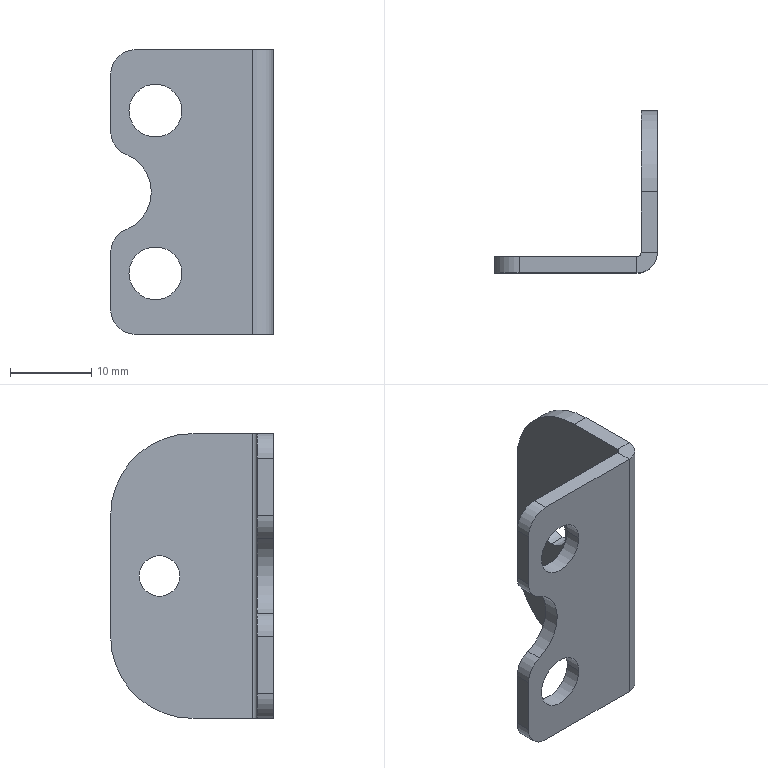Component | SolidWorks | FilmTensionPlate-2 | 1 solid | 28 faces | box 20 x 20 x 35 mm | volume 2267 mm3 | cylinder 15 | plane 13 | commonest cylinder face diameters 6.5 x4 6 x4 5 x3 20 x2 1 x1 10 x1
STEP:
#1=COLOUR_RGB('',0.7922,0.8196,0.9333);
#2=FILL_AREA_STYLE_COLOUR('',#1);
#3=FILL_AREA_STYLE('',(#2));
#4=SURFACE_STYLE_FILL_AREA(#3);
#5=SURFACE_SIDE_STYLE('',(#4));
#6=SURFACE_STYLE_USAGE(.BOTH.,#5);
#7=PRESENTATION_STYLE_ASSIGNMENT((#6));
#8=CARTESIAN_POINT('',(0.9154,-5.709,0.3937));
#9=VERTEX_POINT('',#8);
#10=CARTESIAN_POINT('',(0.6594,-5.709,0.3937));
#11=VERTEX_POINT('',#10);
#12=CARTESIAN_POINT('',(0.7874,-5.709,0.3937));
#13=DIRECTION('',(0.,-1.,0.));
#14=DIRECTION('',(-1.,0.,0.));
#15=AXIS2_PLACEMENT_3D('',#12,#13,#14);
#16=CIRCLE('',#15,0.128);
#17=EDGE_CURVE('',#9,#11,#16,.T.);
#18=ORIENTED_EDGE('',*,*,#17,.F.);
#19=CARTESIAN_POINT('',(0.9154,-5.787,0.3937));
#20=VERTEX_POINT('',#19);
#21=CARTESIAN_POINT('',(0.9154,-5.709,0.3937));
#22=DIRECTION('',(0.,-1.,0.));
#23=VECTOR('',#22,39.37);
#24=LINE('',#21,#23);
#25=EDGE_CURVE('',#9,#20,#24,.T.);
#26=ORIENTED_EDGE('',*,*,#25,.T.);
#27=CARTESIAN_POINT('',(0.6594,-5.787,0.3937));
#28=VERTEX_POINT('',#27);
#29=CARTESIAN_POINT('',(0.7874,-5.787,0.3937));
#30=DIRECTION('',(0.,-1.,0.));
#31=DIRECTION('',(-1.,0.,0.));
#32=AXIS2_PLACEMENT_3D('',#29,#30,#31);
#33=CIRCLE('',#32,0.128);
#34=EDGE_CURVE('',#20,#28,#33,.T.);
#35=ORIENTED_EDGE('',*,*,#34,.T.);
#36=CARTESIAN_POINT('',(0.6594,-5.709,0.3937));
#37=DIRECTION('',(0.,-1.,0.));
#38=VECTOR('',#37,39.37);
#39=LINE('',#36,#38);
#40=EDGE_CURVE('',#11,#28,#39,.T.);
#41=ORIENTED_EDGE('',*,*,#40,.F.);
#42=EDGE_LOOP('',(#18,#26,#35,#41));
#43=FACE_OUTER_BOUND('',#42,.T.);
#44=CARTESIAN_POINT('',(0.7874,-5.709,0.3937));
#45=DIRECTION('',(0.,-1.,0.));
#46=DIRECTION('',(-1.,0.,0.));
#47=AXIS2_PLACEMENT_3D('',#44,#45,#46);
#48=CYLINDRICAL_SURFACE('',#47,0.128);
#49=ADVANCED_FACE('',(#43),#48,.F.);
#50=CARTESIAN_POINT('',(0.9154,-5.709,-0.3937));
#51=VERTEX_POINT('',#50);
#52=CARTESIAN_POINT('',(0.6594,-5.709,-0.3937));
#53=VERTEX_POINT('',#52);
#54=CARTESIAN_POINT('',(0.7874,-5.709,-0.3937));
#55=DIRECTION('',(0.,-1.,0.));
#56=DIRECTION('',(1.,0.,0.));
#57=AXIS2_PLACEMENT_3D('',#54,#55,#56);
#58=CIRCLE('',#57,0.128);
#59=EDGE_CURVE('',#51,#53,#58,.T.);
#60=ORIENTED_EDGE('',*,*,#59,.F.);
#61=CARTESIAN_POINT('',(0.9154,-5.787,-0.3937));
#62=VERTEX_POINT('',#61);
#63=CARTESIAN_POINT('',(0.9154,-5.709,-0.3937));
#64=DIRECTION('',(0.,-1.,0.));
#65=VECTOR('',#64,39.37);
#66=LINE('',#63,#65);
#67=EDGE_CURVE('',#51,#62,#66,.T.);
#68=ORIENTED_EDGE('',*,*,#67,.T.);
#69=CARTESIAN_POINT('',(0.6594,-5.787,-0.3937));
#70=VERTEX_POINT('',#69);
#71=CARTESIAN_POINT('',(0.7874,-5.787,-0.3937));
#72=DIRECTION('',(0.,-1.,0.));
#73=DIRECTION('',(1.,0.,0.));
#74=AXIS2_PLACEMENT_3D('',#71,#72,#73);
#75=CIRCLE('',#74,0.128);
#76=EDGE_CURVE('',#62,#70,#75,.T.);
#77=ORIENTED_EDGE('',*,*,#76,.T.);
#78=CARTESIAN_POINT('',(0.6594,-5.709,-0.3937));
#79=DIRECTION('',(0.,-1.,0.));
#80=VECTOR('',#79,39.37);
#81=LINE('',#78,#80);
#82=EDGE_CURVE('',#53,#70,#81,.T.);
#83=ORIENTED_EDGE('',*,*,#82,.F.);
#84=EDGE_LOOP('',(#60,#68,#77,#83));
#85=FACE_OUTER_BOUND('',#84,.T.);
#86=CARTESIAN_POINT('',(0.7874,-5.709,-0.3937));
#87=DIRECTION('',(0.,-1.,0.));
#88=DIRECTION('',(-1.,0.,0.));
#89=AXIS2_PLACEMENT_3D('',#86,#87,#88);
#90=CYLINDRICAL_SURFACE('',#89,0.128);
#91=ADVANCED_FACE('',(#85),#90,.F.);
#92=CARTESIAN_POINT('',(1.28,-5.236,0.09843));
#93=VERTEX_POINT('',#92);
#94=CARTESIAN_POINT('',(1.28,-5.236,-0.09843));
#95=VERTEX_POINT('',#94);
#96=CARTESIAN_POINT('',(1.28,-5.236,0.));
#97=DIRECTION('',(1.,-0.,0.));
#98=DIRECTION('',(0.,0.,-1.));
#99=AXIS2_PLACEMENT_3D('',#96,#97,#98);
#100=CIRCLE('',#99,0.09843);
#101=EDGE_CURVE('',#93,#95,#100,.T.);
#102=ORIENTED_EDGE('',*,*,#101,.F.);
#103=CARTESIAN_POINT('',(1.358,-5.236,0.09843));
#104=VERTEX_POINT('',#103);
#105=CARTESIAN_POINT('',(1.358,-5.236,0.09843));
#106=DIRECTION('',(1.,-0.,0.));
#107=VECTOR('',#106,39.37);
#108=LINE('',#105,#107);
#109=EDGE_CURVE('',#93,#104,#108,.T.);
#110=ORIENTED_EDGE('',*,*,#109,.T.);
#111=CARTESIAN_POINT('',(1.358,-5.236,-0.09843));
#112=VERTEX_POINT('',#111);
#113=CARTESIAN_POINT('',(1.358,-5.236,0.));
#114=DIRECTION('',(1.,-0.,0.));
#115=DIRECTION('',(0.,0.,-1.));
#116=AXIS2_PLACEMENT_3D('',#113,#114,#115);
#117=CIRCLE('',#116,0.09843);
#118=EDGE_CURVE('',#104,#112,#117,.T.);
#119=ORIENTED_EDGE('',*,*,#118,.T.);
#120=CARTESIAN_POINT('',(1.358,-5.236,-0.09843));
#121=DIRECTION('',(1.,-0.,0.));
#122=VECTOR('',#121,39.37);
#123=LINE('',#120,#122);
#124=EDGE_CURVE('',#95,#112,#123,.T.);
#125=ORIENTED_EDGE('',*,*,#124,.F.);
#126=EDGE_LOOP('',(#102,#110,#119,#125));
#127=FACE_OUTER_BOUND('',#126,.T.);
#128=CARTESIAN_POINT('',(1.358,-5.236,0.));
#129=DIRECTION('',(1.,-0.,0.));
#130=DIRECTION('',(0.,0.,-1.));
#131=AXIS2_PLACEMENT_3D('',#128,#129,#130);
#132=CYLINDRICAL_SURFACE('',#131,0.09843);
#133=ADVANCED_FACE('',(#127),#132,.F.);
#134=CARTESIAN_POINT('',(0.5709,-5.709,0.5709));
#135=VERTEX_POINT('',#134);
#136=CARTESIAN_POINT('',(0.5709,-5.709,0.292));
#137=VERTEX_POINT('',#136);
#138=CARTESIAN_POINT('',(0.5709,-5.709,-0.689));
#139=DIRECTION('',(0.,-0.,-1.));
#140=VECTOR('',#139,39.37);
#141=LINE('',#138,#140);
#142=EDGE_CURVE('',#135,#137,#141,.T.);
#143=ORIENTED_EDGE('',*,*,#142,.T.);
#144=CARTESIAN_POINT('',(0.5709,-5.787,0.292));
#145=VERTEX_POINT('',#144);
#146=CARTESIAN_POINT('',(0.5709,-5.787,0.292));
#147=DIRECTION('',(0.,-1.,0.));
#148=VECTOR('',#147,39.37);
#149=LINE('',#146,#148);
#150=EDGE_CURVE('',#137,#145,#149,.T.);
#151=ORIENTED_EDGE('',*,*,#150,.T.);
#152=CARTESIAN_POINT('',(0.5709,-5.787,0.5709));
#153=VERTEX_POINT('',#152);
#154=CARTESIAN_POINT('',(0.5709,-5.787,0.));
#155=DIRECTION('',(0.,-0.,-1.));
#156=VECTOR('',#155,39.37);
#157=LINE('',#154,#156);
#158=EDGE_CURVE('',#153,#145,#157,.T.);
#159=ORIENTED_EDGE('',*,*,#158,.F.);
#160=CARTESIAN_POINT('',(0.5709,-5.787,0.5709));
#161=DIRECTION('',(-0.,1.,-0.));
#162=VECTOR('',#161,39.37);
#163=LINE('',#160,#162);
#164=EDGE_CURVE('',#153,#135,#163,.T.);
#165=ORIENTED_EDGE('',*,*,#164,.T.);
#166=EDGE_LOOP('',(#143,#151,#159,#165));
#167=FACE_OUTER_BOUND('',#166,.T.);
#168=CARTESIAN_POINT('',(0.5709,-5.787,-0.689));
#169=DIRECTION('',(1.,0.,-0.));
#170=DIRECTION('',(0.,-1.,0.));
#171=AXIS2_PLACEMENT_3D('',#168,#169,#170);
#172=PLANE('',#171);
#173=ADVANCED_FACE('',(#167),#172,.F.);
#174=CARTESIAN_POINT('',(1.358,-5.394,0.689));
#175=VERTEX_POINT('',#174);
#176=CARTESIAN_POINT('',(1.358,-5.689,0.689));
#177=VERTEX_POINT('',#176);
#178=CARTESIAN_POINT('',(1.358,-5.,0.689));
#179=DIRECTION('',(-0.,-1.,0.));
#180=VECTOR('',#179,39.37);
#181=LINE('',#178,#180);
#182=EDGE_CURVE('',#175,#177,#181,.T.);
#183=ORIENTED_EDGE('',*,*,#182,.F.);
#184=CARTESIAN_POINT('',(1.28,-5.394,0.689));
#185=VERTEX_POINT('',#184);
#186=CARTESIAN_POINT('',(1.28,-5.394,0.689));
#187=DIRECTION('',(-1.,0.,-0.));
#188=VECTOR('',#187,39.37);
#189=LINE('',#186,#188);
#190=EDGE_CURVE('',#175,#185,#189,.T.);
#191=ORIENTED_EDGE('',*,*,#190,.T.);
#192=CARTESIAN_POINT('',(1.28,-5.689,0.689));
#193=VERTEX_POINT('',#192);
#194=CARTESIAN_POINT('',(1.28,-5.,0.689));
#195=DIRECTION('',(-0.,-1.,0.));
#196=VECTOR('',#195,39.37);
#197=LINE('',#194,#196);
#198=EDGE_CURVE('',#185,#193,#197,.T.);
#199=ORIENTED_EDGE('',*,*,#198,.T.);
#200=CARTESIAN_POINT('',(1.28,-5.689,0.689));
#201=DIRECTION('',(1.,-0.,0.));
#202=VECTOR('',#201,39.37);
#203=LINE('',#200,#202);
#204=EDGE_CURVE('',#193,#177,#203,.T.);
#205=ORIENTED_EDGE('',*,*,#204,.T.);
#206=EDGE_LOOP('',(#183,#191,#199,#205));
#207=FACE_OUTER_BOUND('',#206,.T.);
#208=CARTESIAN_POINT('',(1.28,-5.,0.689));
#209=DIRECTION('',(-0.,0.,1.));
#210=DIRECTION('',(-0.,-1.,0.));
#211=AXIS2_PLACEMENT_3D('',#208,#209,#210);
#212=PLANE('',#211);
#213=ADVANCED_FACE('',(#207),#212,.T.);
#214=CARTESIAN_POINT('',(1.28,-5.236,0.));
#215=DIRECTION('',(1.,-0.,0.));
#216=DIRECTION('',(0.,0.,-1.));
#217=AXIS2_PLACEMENT_3D('',#214,#215,#216);
#218=CIRCLE('',#217,0.09843);
#219=EDGE_CURVE('',#95,#93,#218,.T.);
#220=ORIENTED_EDGE('',*,*,#219,.T.);
#221=ORIENTED_EDGE('',*,*,#101,.T.);
#222=EDGE_LOOP('',(#220,#221));
#223=FACE_BOUND('',#222,.T.);
#224=CARTESIAN_POINT('',(1.28,-5.,-0.2953));
#225=VERTEX_POINT('',#224);
#226=CARTESIAN_POINT('',(1.28,-5.,0.2953));
#227=VERTEX_POINT('',#226);
#228=CARTESIAN_POINT('',(1.28,-5.,0.689));
#229=DIRECTION('',(0.,0.,1.));
#230=VECTOR('',#229,39.37);
#231=LINE('',#228,#230);
#232=EDGE_CURVE('',#225,#227,#231,.T.);
#233=ORIENTED_EDGE('',*,*,#232,.F.);
#234=CARTESIAN_POINT('',(1.28,-5.394,-0.689));
#235=VERTEX_POINT('',#234);
#236=CARTESIAN_POINT('',(1.28,-5.394,-0.2953));
#237=DIRECTION('',(-1.,0.,-0.));
#238=DIRECTION('',(0.,0.,-1.));
#239=AXIS2_PLACEMENT_3D('',#236,#237,#238);
#240=CIRCLE('',#239,0.3937);
#241=EDGE_CURVE('',#225,#235,#240,.T.);
#242=ORIENTED_EDGE('',*,*,#241,.T.);
#243=CARTESIAN_POINT('',(1.28,-5.689,-0.689));
#244=VERTEX_POINT('',#243);
#245=CARTESIAN_POINT('',(1.28,-5.,-0.689));
#246=DIRECTION('',(0.,1.,-0.));
#247=VECTOR('',#246,39.37);
#248=LINE('',#245,#247);
#249=EDGE_CURVE('',#244,#235,#248,.T.);
#250=ORIENTED_EDGE('',*,*,#249,.F.);
#251=CARTESIAN_POINT('',(1.28,-5.689,0.689));
#252=DIRECTION('',(0.,-0.,-1.));
#253=VECTOR('',#252,39.37);
#254=LINE('',#251,#253);
#255=EDGE_CURVE('',#193,#244,#254,.T.);
#256=ORIENTED_EDGE('',*,*,#255,.F.);
#257=ORIENTED_EDGE('',*,*,#198,.F.);
#258=CARTESIAN_POINT('',(1.28,-5.394,0.2953));
#259=DIRECTION('',(-1.,0.,-0.));
#260=DIRECTION('',(0.,0.,-1.));
#261=AXIS2_PLACEMENT_3D('',#258,#259,#260);
#262=CIRCLE('',#261,0.3937);
#263=EDGE_CURVE('',#185,#227,#262,.T.);
#264=ORIENTED_EDGE('',*,*,#263,.T.);
#265=EDGE_LOOP('',(#233,#242,#250,#256,#257,#264));
#266=FACE_OUTER_BOUND('',#265,.T.);
#267=CARTESIAN_POINT('',(1.28,-5.394,0.));
#268=DIRECTION('',(1.,-0.,0.));
#269=DIRECTION('',(0.,-0.,-1.));
#270=AXIS2_PLACEMENT_3D('',#267,#268,#269);
#271=PLANE('',#270);
#272=ADVANCED_FACE('',(#223,#266),#271,.F.);
#273=CARTESIAN_POINT('',(1.358,-5.236,0.));
#274=DIRECTION('',(1.,-0.,0.));
#275=DIRECTION('',(0.,0.,-1.));
#276=AXIS2_PLACEMENT_3D('',#273,#274,#275);
#277=CIRCLE('',#276,0.09843);
#278=EDGE_CURVE('',#112,#104,#277,.T.);
#279=ORIENTED_EDGE('',*,*,#278,.F.);
#280=ORIENTED_EDGE('',*,*,#118,.F.);
#281=EDGE_LOOP('',(#279,#280));
#282=FACE_BOUND('',#281,.T.);
#283=CARTESIAN_POINT('',(1.358,-5.689,-0.689));
#284=VERTEX_POINT('',#283);
#285=CARTESIAN_POINT('',(1.358,-5.394,-0.689));
#286=VERTEX_POINT('',#285);
#287=CARTESIAN_POINT('',(1.358,-5.,-0.689));
#288=DIRECTION('',(0.,1.,-0.));
#289=VECTOR('',#288,39.37);
#290=LINE('',#287,#289);
#291=EDGE_CURVE('',#284,#286,#290,.T.);
#292=ORIENTED_EDGE('',*,*,#291,.T.);
#293=CARTESIAN_POINT('',(1.358,-5.,-0.2953));
#294=VERTEX_POINT('',#293);
#295=CARTESIAN_POINT('',(1.358,-5.394,-0.2953));
#296=DIRECTION('',(1.,-0.,0.));
#297=DIRECTION('',(0.,0.,-1.));
#298=AXIS2_PLACEMENT_3D('',#295,#296,#297);
#299=CIRCLE('',#298,0.3937);
#300=EDGE_CURVE('',#286,#294,#299,.T.);
#301=ORIENTED_EDGE('',*,*,#300,.T.);
#302=CARTESIAN_POINT('',(1.358,-5.,0.2953));
#303=VERTEX_POINT('',#302);
#304=CARTESIAN_POINT('',(1.358,-5.,0.689));
#305=DIRECTION('',(0.,0.,1.));
#306=VECTOR('',#305,39.37);
#307=LINE('',#304,#306);
#308=EDGE_CURVE('',#294,#303,#307,.T.);
#309=ORIENTED_EDGE('',*,*,#308,.T.);
#310=CARTESIAN_POINT('',(1.358,-5.394,0.2953));
#311=DIRECTION('',(1.,-0.,0.));
#312=DIRECTION('',(0.,0.,-1.));
#313=AXIS2_PLACEMENT_3D('',#310,#311,#312);
#314=CIRCLE('',#313,0.3937);
#315=EDGE_CURVE('',#303,#175,#314,.T.);
#316=ORIENTED_EDGE('',*,*,#315,.T.);
#317=ORIENTED_EDGE('',*,*,#182,.T.);
#318=CARTESIAN_POINT('',(1.358,-5.689,0.689));
#319=DIRECTION('',(0.,-0.,-1.));
#320=VECTOR('',#319,39.37);
#321=LINE('',#318,#320);
#322=EDGE_CURVE('',#177,#284,#321,.T.);
#323=ORIENTED_EDGE('',*,*,#322,.T.);
#324=EDGE_LOOP('',(#292,#301,#309,#316,#317,#323));
#325=FACE_OUTER_BOUND('',#324,.T.);
#326=CARTESIAN_POINT('',(1.358,-5.394,0.));
#327=DIRECTION('',(1.,-0.,0.));
#328=DIRECTION('',(0.,-0.,-1.));
#329=AXIS2_PLACEMENT_3D('',#326,#327,#328);
#330=PLANE('',#329);
#331=ADVANCED_FACE('',(#282,#325),#330,.T.);
#332=ORIENTED_EDGE('',*,*,#249,.T.);
#333=CARTESIAN_POINT('',(1.28,-5.394,-0.689));
#334=DIRECTION('',(1.,-0.,0.));
#335=VECTOR('',#334,39.37);
#336=LINE('',#333,#335);
#337=EDGE_CURVE('',#235,#286,#336,.T.);
#338=ORIENTED_EDGE('',*,*,#337,.T.);
#339=ORIENTED_EDGE('',*,*,#291,.F.);
#340=CARTESIAN_POINT('',(1.28,-5.689,-0.689));
#341=DIRECTION('',(1.,-0.,0.));
#342=VECTOR('',#341,39.37);
#343=LINE('',#340,#342);
#344=EDGE_CURVE('',#244,#284,#343,.T.);
#345=ORIENTED_EDGE('',*,*,#344,.F.);
#346=EDGE_LOOP('',(#332,#338,#339,#345));
#347=FACE_OUTER_BOUND('',#346,.T.);
#348=CARTESIAN_POINT('',(1.28,-5.,-0.689));
#349=DIRECTION('',(0.,-0.,-1.));
#350=DIRECTION('',(0.,1.,-0.));
#351=AXIS2_PLACEMENT_3D('',#348,#349,#350);
#352=PLANE('',#351);
#353=ADVANCED_FACE('',(#347),#352,.T.);
#354=ORIENTED_EDGE('',*,*,#308,.F.);
#355=CARTESIAN_POINT('',(1.28,-5.,-0.2953));
#356=DIRECTION('',(-1.,0.,-0.));
#357=VECTOR('',#356,39.37);
#358=LINE('',#355,#357);
#359=EDGE_CURVE('',#294,#225,#358,.T.);
#360=ORIENTED_EDGE('',*,*,#359,.T.);
#361=ORIENTED_EDGE('',*,*,#232,.T.);
#362=CARTESIAN_POINT('',(1.28,-5.,0.2953));
#363=DIRECTION('',(1.,-0.,0.));
#364=VECTOR('',#363,39.37);
#365=LINE('',#362,#364);
#366=EDGE_CURVE('',#227,#303,#365,.T.);
#367=ORIENTED_EDGE('',*,*,#366,.T.);
#368=EDGE_LOOP('',(#354,#360,#361,#367));
#369=FACE_OUTER_BOUND('',#368,.T.);
#370=CARTESIAN_POINT('',(1.28,-5.,0.689));
#371=DIRECTION('',(0.,1.,-0.));
#372=DIRECTION('',(1.,-0.,0.));
#373=AXIS2_PLACEMENT_3D('',#370,#371,#372);
#374=PLANE('',#373);
#375=ADVANCED_FACE('',(#369),#374,.T.);
#376=CARTESIAN_POINT('',(1.26,-5.709,-0.689));
#377=VERTEX_POINT('',#376);
#378=CARTESIAN_POINT('',(1.26,-5.787,-0.689));
#379=VERTEX_POINT('',#378);
#380=CARTESIAN_POINT('',(1.26,-5.787,-0.689));
#381=DIRECTION('',(0.,-1.,0.));
#382=VECTOR('',#381,39.37);
#383=LINE('',#380,#382);
#384=EDGE_CURVE('',#377,#379,#383,.T.);
#385=ORIENTED_EDGE('',*,*,#384,.F.);
#386=CARTESIAN_POINT('',(1.26,-5.689,-0.689));
#387=DIRECTION('',(0.,-0.,-1.));
#388=DIRECTION('',(1.,0.,0.));
#389=AXIS2_PLACEMENT_3D('',#386,#387,#388);
#390=CIRCLE('',#389,0.01969);
#391=EDGE_CURVE('',#244,#377,#390,.T.);
#392=ORIENTED_EDGE('',*,*,#391,.F.);
#393=ORIENTED_EDGE('',*,*,#344,.T.);
#394=CARTESIAN_POINT('',(1.26,-5.689,-0.689));
#395=DIRECTION('',(0.,-0.,-1.));
#396=DIRECTION('',(1.,-0.,0.));
#397=AXIS2_PLACEMENT_3D('',#394,#395,#396);
#398=CIRCLE('',#397,0.09843);
#399=EDGE_CURVE('',#284,#379,#398,.T.);
#400=ORIENTED_EDGE('',*,*,#399,.T.);
#401=EDGE_LOOP('',(#385,#392,#393,#400));
#402=FACE_OUTER_BOUND('',#401,.T.);
#403=CARTESIAN_POINT('',(1.26,-5.689,-0.689));
#404=DIRECTION('',(0.,-0.,-1.));
#405=DIRECTION('',(-1.,0.,-0.));
#406=AXIS2_PLACEMENT_3D('',#403,#404,#405);
#407=PLANE('',#406);
#408=ADVANCED_FACE('',(#402),#407,.T.);
#409=CARTESIAN_POINT('',(1.26,-5.709,0.689));
#410=VERTEX_POINT('',#409);
#411=CARTESIAN_POINT('',(1.26,-5.689,0.689));
#412=DIRECTION('',(0.,0.,1.));
#413=DIRECTION('',(1.,0.,0.));
#414=AXIS2_PLACEMENT_3D('',#411,#412,#413);
#415=CIRCLE('',#414,0.01969);
#416=EDGE_CURVE('',#410,#193,#415,.T.);
#417=ORIENTED_EDGE('',*,*,#416,.F.);
#418=CARTESIAN_POINT('',(1.26,-5.787,0.689));
#419=VERTEX_POINT('',#418);
#420=CARTESIAN_POINT('',(1.26,-5.709,0.689));
#421=DIRECTION('',(0.,-1.,0.));
#422=VECTOR('',#421,39.37);
#423=LINE('',#420,#422);
#424=EDGE_CURVE('',#410,#419,#423,.T.);
#425=ORIENTED_EDGE('',*,*,#424,.T.);
#426=CARTESIAN_POINT('',(1.26,-5.689,0.689));
#427=DIRECTION('',(0.,0.,1.));
#428=DIRECTION('',(1.,0.,0.));
#429=AXIS2_PLACEMENT_3D('',#426,#427,#428);
#430=CIRCLE('',#429,0.09843);
#431=EDGE_CURVE('',#419,#177,#430,.T.);
#432=ORIENTED_EDGE('',*,*,#431,.T.);
#433=ORIENTED_EDGE('',*,*,#204,.F.);
#434=EDGE_LOOP('',(#417,#425,#432,#433));
#435=FACE_OUTER_BOUND('',#434,.T.);
#436=CARTESIAN_POINT('',(1.26,-5.689,0.689));
#437=DIRECTION('',(0.,-0.,-1.));
#438=DIRECTION('',(-1.,0.,-0.));
#439=AXIS2_PLACEMENT_3D('',#436,#437,#438);
#440=PLANE('',#439);
#441=ADVANCED_FACE('',(#435),#440,.F.);
#442=ORIENTED_EDGE('',*,*,#322,.F.);
#443=ORIENTED_EDGE('',*,*,#431,.F.);
#444=CARTESIAN_POINT('',(1.26,-5.787,-0.689));
#445=DIRECTION('',(0.,-0.,-1.));
#446=VECTOR('',#445,39.37);
#447=LINE('',#444,#446);
#448=EDGE_CURVE('',#419,#379,#447,.T.);
#449=ORIENTED_EDGE('',*,*,#448,.T.);
#450=ORIENTED_EDGE('',*,*,#399,.F.);
#451=EDGE_LOOP('',(#442,#443,#449,#450));
#452=FACE_OUTER_BOUND('',#451,.T.);
#453=CARTESIAN_POINT('',(1.26,-5.689,0.689));
#454=DIRECTION('',(0.,0.,1.));
#455=DIRECTION('',(0.,-1.,0.));
#456=AXIS2_PLACEMENT_3D('',#453,#454,#455);
#457=CYLINDRICAL_SURFACE('',#456,0.09843);
#458=ADVANCED_FACE('',(#452),#457,.T.);
#459=ORIENTED_EDGE('',*,*,#255,.T.);
#460=ORIENTED_EDGE('',*,*,#391,.T.);
#461=CARTESIAN_POINT('',(1.26,-5.709,-0.689));
#462=DIRECTION('',(0.,0.,1.));
#463=VECTOR('',#462,39.37);
#464=LINE('',#461,#463);
#465=EDGE_CURVE('',#377,#410,#464,.T.);
#466=ORIENTED_EDGE('',*,*,#465,.T.);
#467=ORIENTED_EDGE('',*,*,#416,.T.);
#468=EDGE_LOOP('',(#459,#460,#466,#467));
#469=FACE_OUTER_BOUND('',#468,.T.);
#470=CARTESIAN_POINT('',(1.26,-5.689,0.689));
#471=DIRECTION('',(0.,0.,1.));
#472=DIRECTION('',(0.,-1.,0.));
#473=AXIS2_PLACEMENT_3D('',#470,#471,#472);
#474=CYLINDRICAL_SURFACE('',#473,0.01969);
#475=ADVANCED_FACE('',(#469),#474,.F.);
#476=CARTESIAN_POINT('',(0.689,-5.709,0.689));
#477=VERTEX_POINT('',#476);
#478=CARTESIAN_POINT('',(0.5709,-5.709,0.689));
#479=DIRECTION('',(-1.,-0.,-0.));
#480=VECTOR('',#479,39.37);
#481=LINE('',#478,#480);
#482=EDGE_CURVE('',#410,#477,#481,.T.);
#483=ORIENTED_EDGE('',*,*,#482,.T.);
#484=CARTESIAN_POINT('',(0.689,-5.787,0.689));
#485=VERTEX_POINT('',#484);
#486=CARTESIAN_POINT('',(0.689,-5.787,0.689));
#487=DIRECTION('',(0.,-1.,0.));
#488=VECTOR('',#487,39.37);
#489=LINE('',#486,#488);
#490=EDGE_CURVE('',#477,#485,#489,.T.);
#491=ORIENTED_EDGE('',*,*,#490,.T.);
#492=CARTESIAN_POINT('',(1.358,-5.787,0.689));
#493=DIRECTION('',(-1.,-0.,-0.));
#494=VECTOR('',#493,39.37);
#495=LINE('',#492,#494);
#496=EDGE_CURVE('',#419,#485,#495,.T.);
#497=ORIENTED_EDGE('',*,*,#496,.F.);
#498=ORIENTED_EDGE('',*,*,#424,.F.);
#499=EDGE_LOOP('',(#483,#491,#497,#498));
#500=FACE_OUTER_BOUND('',#499,.T.);
#501=CARTESIAN_POINT('',(0.5709,-5.787,0.689));
#502=DIRECTION('',(0.,-0.,-1.));
#503=DIRECTION('',(-1.,0.,-0.));
#504=AXIS2_PLACEMENT_3D('',#501,#502,#503);
#505=PLANE('',#504);
#506=ADVANCED_FACE('',(#500),#505,.F.);
#507=CARTESIAN_POINT('',(0.689,-5.787,-0.689));
#508=VERTEX_POINT('',#507);
#509=CARTESIAN_POINT('',(1.358,-5.787,-0.689));
#510=DIRECTION('',(1.,0.,-0.));
#511=VECTOR('',#510,39.37);
#512=LINE('',#509,#511);
#513=EDGE_CURVE('',#508,#379,#512,.T.);
#514=ORIENTED_EDGE('',*,*,#513,.F.);
#515=CARTESIAN_POINT('',(0.689,-5.709,-0.689));
#516=VERTEX_POINT('',#515);
#517=CARTESIAN_POINT('',(0.689,-5.787,-0.689));
#518=DIRECTION('',(-0.,1.,-0.));
#519=VECTOR('',#518,39.37);
#520=LINE('',#517,#519);
#521=EDGE_CURVE('',#508,#516,#520,.T.);
#522=ORIENTED_EDGE('',*,*,#521,.T.);
#523=CARTESIAN_POINT('',(1.28,-5.709,-0.689));
#524=DIRECTION('',(1.,0.,-0.));
#525=VECTOR('',#524,39.37);
#526=LINE('',#523,#525);
#527=EDGE_CURVE('',#516,#377,#526,.T.);
#528=ORIENTED_EDGE('',*,*,#527,.T.);
#529=ORIENTED_EDGE('',*,*,#384,.T.);
#530=EDGE_LOOP('',(#514,#522,#528,#529));
#531=FACE_OUTER_BOUND('',#530,.T.);
#532=CARTESIAN_POINT('',(1.28,-5.787,-0.689));
#533=DIRECTION('',(-0.,0.,1.));
#534=DIRECTION('',(1.,-0.,0.));
#535=AXIS2_PLACEMENT_3D('',#532,#533,#534);
#536=PLANE('',#535);
#537=ADVANCED_FACE('',(#531),#536,.F.);
#538=CARTESIAN_POINT('',(0.7874,-5.787,0.3937));
#539=DIRECTION('',(0.,-1.,0.));
#540=DIRECTION('',(-1.,0.,0.));
#541=AXIS2_PLACEMENT_3D('',#538,#539,#540);
#542=CIRCLE('',#541,0.128);
#543=EDGE_CURVE('',#28,#20,#542,.T.);
#544=ORIENTED_EDGE('',*,*,#543,.F.);
#545=ORIENTED_EDGE('',*,*,#34,.F.);
#546=EDGE_LOOP('',(#544,#545));
#547=FACE_BOUND('',#546,.T.);
#548=CARTESIAN_POINT('',(0.7874,-5.787,-0.3937));
#549=DIRECTION('',(0.,-1.,0.));
#550=DIRECTION('',(1.,0.,0.));
#551=AXIS2_PLACEMENT_3D('',#548,#549,#550);
#552=CIRCLE('',#551,0.128);
#553=EDGE_CURVE('',#70,#62,#552,.T.);
#554=ORIENTED_EDGE('',*,*,#553,.F.);
#555=ORIENTED_EDGE('',*,*,#76,.F.);
#556=EDGE_LOOP('',(#554,#555));
#557=FACE_BOUND('',#556,.T.);
#558=CARTESIAN_POINT('',(0.5709,-5.787,-0.292));
#559=VERTEX_POINT('',#558);
#560=CARTESIAN_POINT('',(0.5709,-5.787,-0.5709));
#561=VERTEX_POINT('',#560);
#562=CARTESIAN_POINT('',(0.5709,-5.787,0.));
#563=DIRECTION('',(0.,-0.,-1.));
#564=VECTOR('',#563,39.37);
#565=LINE('',#562,#564);
#566=EDGE_CURVE('',#559,#561,#565,.T.);
#567=ORIENTED_EDGE('',*,*,#566,.T.);
#568=CARTESIAN_POINT('',(0.689,-5.787,-0.5709));
#569=DIRECTION('',(0.,-1.,0.));
#570=DIRECTION('',(1.,0.,0.));
#571=AXIS2_PLACEMENT_3D('',#568,#569,#570);
#572=CIRCLE('',#571,0.1181);
#573=EDGE_CURVE('',#561,#508,#572,.T.);
#574=ORIENTED_EDGE('',*,*,#573,.T.);
#575=ORIENTED_EDGE('',*,*,#513,.T.);
#576=ORIENTED_EDGE('',*,*,#448,.F.);
#577=ORIENTED_EDGE('',*,*,#496,.T.);
#578=CARTESIAN_POINT('',(0.689,-5.787,0.5709));
#579=DIRECTION('',(0.,-1.,0.));
#580=DIRECTION('',(1.,0.,0.));
#581=AXIS2_PLACEMENT_3D('',#578,#579,#580);
#582=CIRCLE('',#581,0.1181);
#583=EDGE_CURVE('',#485,#153,#582,.T.);
#584=ORIENTED_EDGE('',*,*,#583,.T.);
#585=ORIENTED_EDGE('',*,*,#158,.T.);
#586=CARTESIAN_POINT('',(0.6447,-5.787,0.1825));
#587=VERTEX_POINT('',#586);
#588=CARTESIAN_POINT('',(0.689,-5.787,0.292));
#589=DIRECTION('',(0.,-1.,0.));
#590=DIRECTION('',(1.,0.,0.));
#591=AXIS2_PLACEMENT_3D('',#588,#589,#590);
#592=CIRCLE('',#591,0.1181);
#593=EDGE_CURVE('',#145,#587,#592,.T.);
#594=ORIENTED_EDGE('',*,*,#593,.T.);
#595=CARTESIAN_POINT('',(0.6447,-5.787,-0.1825));
#596=VERTEX_POINT('',#595);
#597=CARTESIAN_POINT('',(0.5709,-5.787,0.));
#598=DIRECTION('',(0.,-1.,0.));
#599=DIRECTION('',(-1.,0.,0.));
#600=AXIS2_PLACEMENT_3D('',#597,#598,#599);
#601=CIRCLE('',#600,0.1969);
#602=EDGE_CURVE('',#596,#587,#601,.T.);
#603=ORIENTED_EDGE('',*,*,#602,.F.);
#604=CARTESIAN_POINT('',(0.689,-5.787,-0.292));
#605=DIRECTION('',(0.,-1.,0.));
#606=DIRECTION('',(1.,0.,-0.));
#607=AXIS2_PLACEMENT_3D('',#604,#605,#606);
#608=CIRCLE('',#607,0.1181);
#609=EDGE_CURVE('',#596,#559,#608,.T.);
#610=ORIENTED_EDGE('',*,*,#609,.T.);
#611=EDGE_LOOP('',(#567,#574,#575,#576,#577,#584,#585,#594,#603,#610));
#612=FACE_OUTER_BOUND('',#611,.T.);
#613=CARTESIAN_POINT('',(1.358,-5.787,0.));
#614=DIRECTION('',(-0.,1.,-0.));
#615=DIRECTION('',(1.,0.,-0.));
#616=AXIS2_PLACEMENT_3D('',#613,#614,#615);
#617=PLANE('',#616);
#618=ADVANCED_FACE('',(#547,#557,#612),#617,.F.);
#619=CARTESIAN_POINT('',(0.7874,-5.709,0.3937));
#620=DIRECTION('',(0.,-1.,0.));
#621=DIRECTION('',(-1.,0.,0.));
#622=AXIS2_PLACEMENT_3D('',#619,#620,#621);
#623=CIRCLE('',#622,0.128);
#624=EDGE_CURVE('',#11,#9,#623,.T.);
#625=ORIENTED_EDGE('',*,*,#624,.T.);
#626=ORIENTED_EDGE('',*,*,#17,.T.);
#627=EDGE_LOOP('',(#625,#626));
#628=FACE_BOUND('',#627,.T.);
#629=CARTESIAN_POINT('',(0.7874,-5.709,-0.3937));
#630=DIRECTION('',(0.,-1.,0.));
#631=DIRECTION('',(1.,0.,0.));
#632=AXIS2_PLACEMENT_3D('',#629,#630,#631);
#633=CIRCLE('',#632,0.128);
#634=EDGE_CURVE('',#53,#51,#633,.T.);
#635=ORIENTED_EDGE('',*,*,#634,.T.);
#636=ORIENTED_EDGE('',*,*,#59,.T.);
#637=EDGE_LOOP('',(#635,#636));
#638=FACE_BOUND('',#637,.T.);
#639=ORIENTED_EDGE('',*,*,#527,.F.);
#640=CARTESIAN_POINT('',(0.5709,-5.709,-0.5709));
#641=VERTEX_POINT('',#640);
#642=CARTESIAN_POINT('',(0.689,-5.709,-0.5709));
#643=DIRECTION('',(-0.,1.,-0.));
#644=DIRECTION('',(1.,0.,0.));
#645=AXIS2_PLACEMENT_3D('',#642,#643,#644);
#646=CIRCLE('',#645,0.1181);
#647=EDGE_CURVE('',#516,#641,#646,.T.);
#648=ORIENTED_EDGE('',*,*,#647,.T.);
#649=CARTESIAN_POINT('',(0.5709,-5.709,-0.292));
#650=VERTEX_POINT('',#649);
#651=CARTESIAN_POINT('',(0.5709,-5.709,-0.689));
#652=DIRECTION('',(0.,-0.,-1.));
#653=VECTOR('',#652,39.37);
#654=LINE('',#651,#653);
#655=EDGE_CURVE('',#650,#641,#654,.T.);
#656=ORIENTED_EDGE('',*,*,#655,.F.);
#657=CARTESIAN_POINT('',(0.6447,-5.709,-0.1825));
#658=VERTEX_POINT('',#657);
#659=CARTESIAN_POINT('',(0.689,-5.709,-0.292));
#660=DIRECTION('',(-0.,1.,-0.));
#661=DIRECTION('',(1.,0.,0.));
#662=AXIS2_PLACEMENT_3D('',#659,#660,#661);
#663=CIRCLE('',#662,0.1181);
#664=EDGE_CURVE('',#650,#658,#663,.T.);
#665=ORIENTED_EDGE('',*,*,#664,.T.);
#666=CARTESIAN_POINT('',(0.6447,-5.709,0.1825));
#667=VERTEX_POINT('',#666);
#668=CARTESIAN_POINT('',(0.5709,-5.709,0.));
#669=DIRECTION('',(0.,-1.,0.));
#670=DIRECTION('',(-1.,0.,0.));
#671=AXIS2_PLACEMENT_3D('',#668,#669,#670);
#672=CIRCLE('',#671,0.1969);
#673=EDGE_CURVE('',#658,#667,#672,.T.);
#674=ORIENTED_EDGE('',*,*,#673,.T.);
#675=CARTESIAN_POINT('',(0.689,-5.709,0.292));
#676=DIRECTION('',(-0.,1.,-0.));
#677=DIRECTION('',(1.,0.,0.));
#678=AXIS2_PLACEMENT_3D('',#675,#676,#677);
#679=CIRCLE('',#678,0.1181);
#680=EDGE_CURVE('',#667,#137,#679,.T.);
#681=ORIENTED_EDGE('',*,*,#680,.T.);
#682=ORIENTED_EDGE('',*,*,#142,.F.);
#683=CARTESIAN_POINT('',(0.689,-5.709,0.5709));
#684=DIRECTION('',(-0.,1.,-0.));
#685=DIRECTION('',(1.,0.,0.));
#686=AXIS2_PLACEMENT_3D('',#683,#684,#685);
#687=CIRCLE('',#686,0.1181);
#688=EDGE_CURVE('',#135,#477,#687,.T.);
#689=ORIENTED_EDGE('',*,*,#688,.T.);
#690=ORIENTED_EDGE('',*,*,#482,.F.);
#691=ORIENTED_EDGE('',*,*,#465,.F.);
#692=EDGE_LOOP('',(#639,#648,#656,#665,#674,#681,#682,#689,#690,#691));
#693=FACE_OUTER_BOUND('',#692,.T.);
#694=CARTESIAN_POINT('',(1.358,-5.709,0.));
#695=DIRECTION('',(-0.,1.,-0.));
#696=DIRECTION('',(1.,0.,-0.));
#697=AXIS2_PLACEMENT_3D('',#694,#695,#696);
#698=PLANE('',#697);
#699=ADVANCED_FACE('',(#628,#638,#693),#698,.T.);
#700=ORIENTED_EDGE('',*,*,#655,.T.);
#701=CARTESIAN_POINT('',(0.5709,-5.787,-0.5709));
#702=DIRECTION('',(0.,-1.,0.));
#703=VECTOR('',#702,39.37);
#704=LINE('',#701,#703);
#705=EDGE_CURVE('',#641,#561,#704,.T.);
#706=ORIENTED_EDGE('',*,*,#705,.T.);
#707=ORIENTED_EDGE('',*,*,#566,.F.);
#708=CARTESIAN_POINT('',(0.5709,-5.787,-0.292));
#709=DIRECTION('',(-0.,1.,-0.));
#710=VECTOR('',#709,39.37);
#711=LINE('',#708,#710);
#712=EDGE_CURVE('',#559,#650,#711,.T.);
#713=ORIENTED_EDGE('',*,*,#712,.T.);
#714=EDGE_LOOP('',(#700,#706,#707,#713));
#715=FACE_OUTER_BOUND('',#714,.T.);
#716=CARTESIAN_POINT('',(0.5709,-5.787,-0.689));
#717=DIRECTION('',(1.,0.,-0.));
#718=DIRECTION('',(0.,-1.,0.));
#719=AXIS2_PLACEMENT_3D('',#716,#717,#718);
#720=PLANE('',#719);
#721=ADVANCED_FACE('',(#715),#720,.F.);
#722=ORIENTED_EDGE('',*,*,#109,.F.);
#723=ORIENTED_EDGE('',*,*,#219,.F.);
#724=ORIENTED_EDGE('',*,*,#124,.T.);
#725=ORIENTED_EDGE('',*,*,#278,.T.);
#726=EDGE_LOOP('',(#722,#723,#724,#725));
#727=FACE_OUTER_BOUND('',#726,.T.);
#728=CARTESIAN_POINT('',(1.358,-5.236,0.));
#729=DIRECTION('',(1.,-0.,0.));
#730=DIRECTION('',(0.,0.,-1.));
#731=AXIS2_PLACEMENT_3D('',#728,#729,#730);
#732=CYLINDRICAL_SURFACE('',#731,0.09843);
#733=ADVANCED_FACE('',(#727),#732,.F.);
#734=ORIENTED_EDGE('',*,*,#241,.F.);
#735=ORIENTED_EDGE('',*,*,#359,.F.);
#736=ORIENTED_EDGE('',*,*,#300,.F.);
#737=ORIENTED_EDGE('',*,*,#337,.F.);
#738=EDGE_LOOP('',(#734,#735,#736,#737));
#739=FACE_OUTER_BOUND('',#738,.T.);
#740=CARTESIAN_POINT('',(1.28,-5.394,-0.2953));
#741=DIRECTION('',(1.,-0.,0.));
#742=DIRECTION('',(0.,0.,-1.));
#743=AXIS2_PLACEMENT_3D('',#740,#741,#742);
#744=CYLINDRICAL_SURFACE('',#743,0.3937);
#745=ADVANCED_FACE('',(#739),#744,.T.);
#746=ORIENTED_EDGE('',*,*,#263,.F.);
#747=ORIENTED_EDGE('',*,*,#190,.F.);
#748=ORIENTED_EDGE('',*,*,#315,.F.);
#749=ORIENTED_EDGE('',*,*,#366,.F.);
#750=EDGE_LOOP('',(#746,#747,#748,#749));
#751=FACE_OUTER_BOUND('',#750,.T.);
#752=CARTESIAN_POINT('',(1.28,-5.394,0.2953));
#753=DIRECTION('',(1.,-0.,0.));
#754=DIRECTION('',(0.,0.,-1.));
#755=AXIS2_PLACEMENT_3D('',#752,#753,#754);
#756=CYLINDRICAL_SURFACE('',#755,0.3937);
#757=ADVANCED_FACE('',(#751),#756,.T.);
#758=ORIENTED_EDGE('',*,*,#673,.F.);
#759=CARTESIAN_POINT('',(0.6447,-5.709,-0.1825));
#760=DIRECTION('',(0.,-1.,0.));
#761=VECTOR('',#760,39.37);
#762=LINE('',#759,#761);
#763=EDGE_CURVE('',#658,#596,#762,.T.);
#764=ORIENTED_EDGE('',*,*,#763,.T.);
#765=ORIENTED_EDGE('',*,*,#602,.T.);
#766=CARTESIAN_POINT('',(0.6447,-5.709,0.1825));
#767=DIRECTION('',(-0.,1.,-0.));
#768=VECTOR('',#767,39.37);
#769=LINE('',#766,#768);
#770=EDGE_CURVE('',#587,#667,#769,.T.);
#771=ORIENTED_EDGE('',*,*,#770,.T.);
#772=EDGE_LOOP('',(#758,#764,#765,#771));
#773=FACE_OUTER_BOUND('',#772,.T.);
#774=CARTESIAN_POINT('',(0.5709,-5.709,0.));
#775=DIRECTION('',(0.,-1.,0.));
#776=DIRECTION('',(-1.,0.,0.));
#777=AXIS2_PLACEMENT_3D('',#774,#775,#776);
#778=CYLINDRICAL_SURFACE('',#777,0.1969);
#779=ADVANCED_FACE('',(#773),#778,.F.);
#780=ORIENTED_EDGE('',*,*,#67,.F.);
#781=ORIENTED_EDGE('',*,*,#634,.F.);
#782=ORIENTED_EDGE('',*,*,#82,.T.);
#783=ORIENTED_EDGE('',*,*,#553,.T.);
#784=EDGE_LOOP('',(#780,#781,#782,#783));
#785=FACE_OUTER_BOUND('',#784,.T.);
#786=CARTESIAN_POINT('',(0.7874,-5.709,-0.3937));
#787=DIRECTION('',(0.,-1.,0.));
#788=DIRECTION('',(-1.,0.,0.));
#789=AXIS2_PLACEMENT_3D('',#786,#787,#788);
#790=CYLINDRICAL_SURFACE('',#789,0.128);
#791=ADVANCED_FACE('',(#785),#790,.F.);
#792=ORIENTED_EDGE('',*,*,#25,.F.);
#793=ORIENTED_EDGE('',*,*,#624,.F.);
#794=ORIENTED_EDGE('',*,*,#40,.T.);
#795=ORIENTED_EDGE('',*,*,#543,.T.);
#796=EDGE_LOOP('',(#792,#793,#794,#795));
#797=FACE_OUTER_BOUND('',#796,.T.);
#798=CARTESIAN_POINT('',(0.7874,-5.709,0.3937));
#799=DIRECTION('',(0.,-1.,0.));
#800=DIRECTION('',(-1.,0.,0.));
#801=AXIS2_PLACEMENT_3D('',#798,#799,#800);
#802=CYLINDRICAL_SURFACE('',#801,0.128);
#803=ADVANCED_FACE('',(#797),#802,.F.);
#804=ORIENTED_EDGE('',*,*,#573,.F.);
#805=ORIENTED_EDGE('',*,*,#705,.F.);
#806=ORIENTED_EDGE('',*,*,#647,.F.);
#807=ORIENTED_EDGE('',*,*,#521,.F.);
#808=EDGE_LOOP('',(#804,#805,#806,#807));
#809=FACE_OUTER_BOUND('',#808,.T.);
#810=CARTESIAN_POINT('',(0.689,-5.787,-0.5709));
#811=DIRECTION('',(-0.,1.,-0.));
#812=DIRECTION('',(1.,0.,0.));
#813=AXIS2_PLACEMENT_3D('',#810,#811,#812);
#814=CYLINDRICAL_SURFACE('',#813,0.1181);
#815=ADVANCED_FACE('',(#809),#814,.T.);
#816=ORIENTED_EDGE('',*,*,#609,.F.);
#817=ORIENTED_EDGE('',*,*,#763,.F.);
#818=ORIENTED_EDGE('',*,*,#664,.F.);
#819=ORIENTED_EDGE('',*,*,#712,.F.);
#820=EDGE_LOOP('',(#816,#817,#818,#819));
#821=FACE_OUTER_BOUND('',#820,.T.);
#822=CARTESIAN_POINT('',(0.689,-5.709,-0.292));
#823=DIRECTION('',(0.,-1.,0.));
#824=DIRECTION('',(-1.,0.,0.));
#825=AXIS2_PLACEMENT_3D('',#822,#823,#824);
#826=CYLINDRICAL_SURFACE('',#825,0.1181);
#827=ADVANCED_FACE('',(#821),#826,.T.);
#828=ORIENTED_EDGE('',*,*,#680,.F.);
#829=ORIENTED_EDGE('',*,*,#770,.F.);
#830=ORIENTED_EDGE('',*,*,#593,.F.);
#831=ORIENTED_EDGE('',*,*,#150,.F.);
#832=EDGE_LOOP('',(#828,#829,#830,#831));
#833=FACE_OUTER_BOUND('',#832,.T.);
#834=CARTESIAN_POINT('',(0.689,-5.709,0.292));
#835=DIRECTION('',(0.,-1.,0.));
#836=DIRECTION('',(-1.,0.,0.));
#837=AXIS2_PLACEMENT_3D('',#834,#835,#836);
#838=CYLINDRICAL_SURFACE('',#837,0.1181);
#839=ADVANCED_FACE('',(#833),#838,.T.);
#840=ORIENTED_EDGE('',*,*,#583,.F.);
#841=ORIENTED_EDGE('',*,*,#490,.F.);
#842=ORIENTED_EDGE('',*,*,#688,.F.);
#843=ORIENTED_EDGE('',*,*,#164,.F.);
#844=EDGE_LOOP('',(#840,#841,#842,#843));
#845=FACE_OUTER_BOUND('',#844,.T.);
#846=CARTESIAN_POINT('',(0.689,-5.787,0.5709));
#847=DIRECTION('',(-0.,1.,-0.));
#848=DIRECTION('',(1.,0.,0.));
#849=AXIS2_PLACEMENT_3D('',#846,#847,#848);
#850=CYLINDRICAL_SURFACE('',#849,0.1181);
#851=ADVANCED_FACE('',(#845),#850,.T.);
#852=CLOSED_SHELL('',(#49,#91,#133,#173,#213,#272,#331,#353,#375,#408,#441,#458,#475,#506,#537,#618,#699,#721,#733,#745,#757,#779,#791,#803,#815,#827,#839,#851));
#853=MANIFOLD_SOLID_BREP('',#852);
#854=STYLED_ITEM('',(#7),#853);
#855=(LENGTH_UNIT()NAMED_UNIT(*)SI_UNIT($,.METRE.));
#856=LENGTH_MEASURE_WITH_UNIT(LENGTH_MEASURE(0.0254),#855);
#857=DIMENSIONAL_EXPONENTS(1.,0.,0.,0.,0.,0.,0.);
#858=(CONVERSION_BASED_UNIT('',#856)LENGTH_UNIT()NAMED_UNIT(#857));
#859=UNCERTAINTY_MEASURE_WITH_UNIT(LENGTH_MEASURE(0.00001),#858,'','');
#860=(NAMED_UNIT(*)PLANE_ANGLE_UNIT()SI_UNIT($,.RADIAN.));
#861=(NAMED_UNIT(*)SI_UNIT($,.STERADIAN.)SOLID_ANGLE_UNIT());
#862=(GEOMETRIC_REPRESENTATION_CONTEXT(3)GLOBAL_UNCERTAINTY_ASSIGNED_CONTEXT((#859))GLOBAL_UNIT_ASSIGNED_CONTEXT((#858,#860,#861))REPRESENTATION_CONTEXT('',''));
#863=MECHANICAL_DESIGN_GEOMETRIC_PRESENTATION_REPRESENTATION('',(#854),#862);
#864=CARTESIAN_POINT('',(0.,0.,0.));
#865=DIRECTION('',(0.,0.,1.));
#866=DIRECTION('',(1.,0.,0.));
#867=AXIS2_PLACEMENT_3D('',#864,#865,#866);
#868=(LENGTH_UNIT()NAMED_UNIT(*)SI_UNIT($,.METRE.));
#869=LENGTH_MEASURE_WITH_UNIT(LENGTH_MEASURE(0.0254),#868);
#870=DIMENSIONAL_EXPONENTS(1.,0.,0.,0.,0.,0.,0.);
#871=(CONVERSION_BASED_UNIT('',#869)LENGTH_UNIT()NAMED_UNIT(#870));
#872=UNCERTAINTY_MEASURE_WITH_UNIT(LENGTH_MEASURE(0.00001),#871,'','');
#873=(NAMED_UNIT(*)PLANE_ANGLE_UNIT()SI_UNIT($,.RADIAN.));
#874=(NAMED_UNIT(*)SI_UNIT($,.STERADIAN.)SOLID_ANGLE_UNIT());
#875=(GEOMETRIC_REPRESENTATION_CONTEXT(3)GLOBAL_UNCERTAINTY_ASSIGNED_CONTEXT((#872))GLOBAL_UNIT_ASSIGNED_CONTEXT((#871,#873,#874))REPRESENTATION_CONTEXT('',''));
#876=ADVANCED_BREP_SHAPE_REPRESENTATION('',(#853,#867),#875);
#877=PRESENTATION_LAYER_ASSIGNMENT('','',(#854));